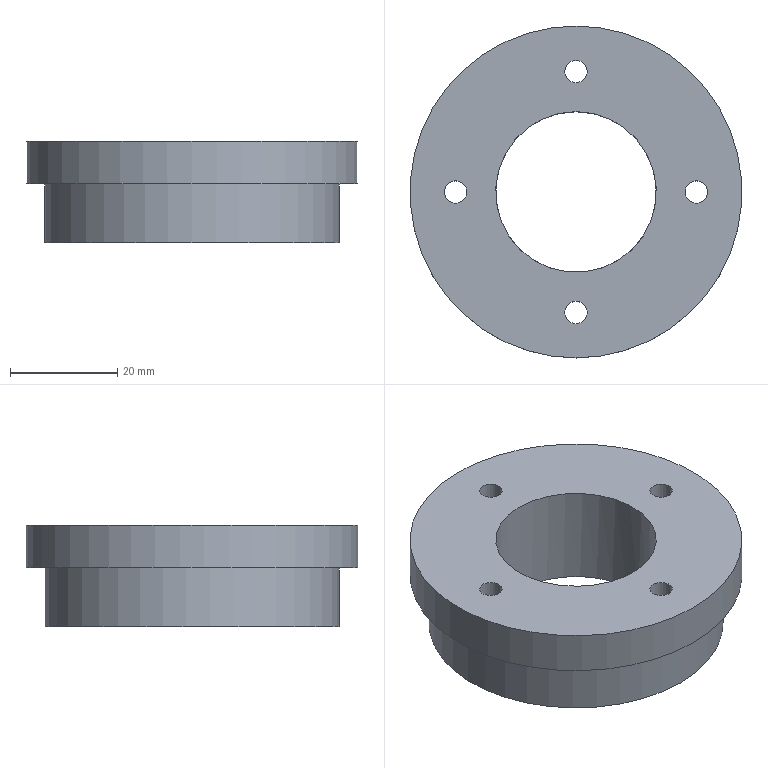Component | NX | FLANGE | 1 solid | 10 faces | box 62 x 62 x 19 mm | volume 35803 mm3 | cylinder 7 | plane 3 | commonest cylinder face diameters 4.2 x4 55 x1 62 x1 30 x1
STEP:
#1=CARTESIAN_POINT('',(0.,0.,0.));
#2=DIRECTION('',(0.,0.,1.));
#3=DIRECTION('',(1.,0.,0.));
#4=AXIS2_PLACEMENT_3D('',#1,#2,#3);
#5=CARTESIAN_POINT('',(0.,-27.5,14.));
#6=VERTEX_POINT('',#5);
#7=CARTESIAN_POINT('',(0.,0.,14.));
#8=DIRECTION('',(0.,0.,1.));
#9=DIRECTION('',(0.,-1.,0.));
#10=AXIS2_PLACEMENT_3D('',#7,#8,#9);
#11=CIRCLE('',#10,27.5);
#12=CARTESIAN_POINT('',(0.,0.,14.));
#13=DIRECTION('',(0.,0.,-1.));
#14=DIRECTION('',(0.,1.,0.));
#15=AXIS2_PLACEMENT_3D('',#12,#13,#14);
#16=CYLINDRICAL_SURFACE('',#15,27.5);
#17=CARTESIAN_POINT('',(9.425,0.));
#18=DIRECTION('',(-1.,0.));
#19=VECTOR('',#18,1.);
#20=LINE('',#17,#19);
#21=(GEOMETRIC_REPRESENTATION_CONTEXT(2)PARAMETRIC_REPRESENTATION_CONTEXT()REPRESENTATION_CONTEXT('',''));
#22=DEFINITIONAL_REPRESENTATION('',(#20),#21);
#23=PCURVE('',#16,#22);
#24=CARTESIAN_POINT('',(0.,0.,14.));
#25=DIRECTION('',(0.,0.,1.));
#26=DIRECTION('',(0.,-1.,0.));
#27=AXIS2_PLACEMENT_3D('',#24,#25,#26);
#28=PLANE('',#27);
#29=CARTESIAN_POINT('',(0.,0.));
#30=DIRECTION('',(1.,0.));
#31=AXIS2_PLACEMENT_2D('',#29,#30);
#32=CIRCLE('',#31,27.5);
#33=(GEOMETRIC_REPRESENTATION_CONTEXT(2)PARAMETRIC_REPRESENTATION_CONTEXT()REPRESENTATION_CONTEXT('',''));
#34=DEFINITIONAL_REPRESENTATION('',(#32),#33);
#35=PCURVE('',#28,#34);
#36=SURFACE_CURVE('',#11,(#23,#35),.PCURVE_S1.);
#37=EDGE_CURVE('',#6,#6,#36,.T.);
#38=ORIENTED_EDGE('',*,*,#37,.F.);
#39=CARTESIAN_POINT('',(0.,-27.5,3.));
#40=VERTEX_POINT('',#39);
#41=CARTESIAN_POINT('',(0.,-27.5,14.));
#42=CARTESIAN_POINT('',(0.,-27.5,3.));
#43=B_SPLINE_CURVE_WITH_KNOTS('',1,(#41,#42),.UNSPECIFIED.,.F.,.F.,(2,2),(0.,11.),.PIECEWISE_BEZIER_KNOTS.);
#44=CARTESIAN_POINT('',(9.425,0.));
#45=DIRECTION('',(0.,1.));
#46=VECTOR('',#45,1.);
#47=LINE('',#44,#46);
#48=(GEOMETRIC_REPRESENTATION_CONTEXT(2)PARAMETRIC_REPRESENTATION_CONTEXT()REPRESENTATION_CONTEXT('',''));
#49=DEFINITIONAL_REPRESENTATION('',(#47),#48);
#50=PCURVE('',#16,#49);
#51=CARTESIAN_POINT('',(3.142,0.));
#52=DIRECTION('',(0.,1.));
#53=VECTOR('',#52,1.);
#54=LINE('',#51,#53);
#55=(GEOMETRIC_REPRESENTATION_CONTEXT(2)PARAMETRIC_REPRESENTATION_CONTEXT()REPRESENTATION_CONTEXT('',''));
#56=DEFINITIONAL_REPRESENTATION('',(#54),#55);
#57=PCURVE('',#16,#56);
#58=SEAM_CURVE('',#43,(#50,#57),.PCURVE_S1.);
#59=EDGE_CURVE('',#6,#40,#58,.T.);
#60=ORIENTED_EDGE('',*,*,#59,.T.);
#61=CARTESIAN_POINT('',(0.,0.,3.));
#62=DIRECTION('',(0.,0.,1.));
#63=DIRECTION('',(0.,-1.,0.));
#64=AXIS2_PLACEMENT_3D('',#61,#62,#63);
#65=CIRCLE('',#64,27.5);
#66=CARTESIAN_POINT('',(9.425,11.));
#67=DIRECTION('',(-1.,0.));
#68=VECTOR('',#67,1.);
#69=LINE('',#66,#68);
#70=(GEOMETRIC_REPRESENTATION_CONTEXT(2)PARAMETRIC_REPRESENTATION_CONTEXT()REPRESENTATION_CONTEXT('',''));
#71=DEFINITIONAL_REPRESENTATION('',(#69),#70);
#72=PCURVE('',#16,#71);
#73=CARTESIAN_POINT('',(0.,0.,3.));
#74=DIRECTION('',(0.,0.,1.));
#75=DIRECTION('',(0.,-1.,0.));
#76=AXIS2_PLACEMENT_3D('',#73,#74,#75);
#77=PLANE('',#76);
#78=CARTESIAN_POINT('',(0.,0.));
#79=DIRECTION('',(1.,0.));
#80=AXIS2_PLACEMENT_2D('',#78,#79);
#81=CIRCLE('',#80,27.5);
#82=(GEOMETRIC_REPRESENTATION_CONTEXT(2)PARAMETRIC_REPRESENTATION_CONTEXT()REPRESENTATION_CONTEXT('',''));
#83=DEFINITIONAL_REPRESENTATION('',(#81),#82);
#84=PCURVE('',#77,#83);
#85=SURFACE_CURVE('',#65,(#72,#84),.PCURVE_S1.);
#86=EDGE_CURVE('',#40,#40,#85,.T.);
#87=ORIENTED_EDGE('',*,*,#86,.T.);
#88=ORIENTED_EDGE('',*,*,#59,.F.);
#89=EDGE_LOOP('',(#38,#60,#87,#88));
#90=FACE_BOUND('',#89,.T.);
#91=ADVANCED_FACE('',(#90),#16,.T.);
#92=CARTESIAN_POINT('',(0.,-24.6,3.));
#93=VERTEX_POINT('',#92);
#94=CARTESIAN_POINT('',(0.,-20.4,3.));
#95=VERTEX_POINT('',#94);
#96=CARTESIAN_POINT('',(0.,-22.5,3.));
#97=DIRECTION('',(0.,0.,1.));
#98=DIRECTION('',(0.,-1.,0.));
#99=AXIS2_PLACEMENT_3D('',#96,#97,#98);
#100=CIRCLE('',#99,2.1);
#101=CARTESIAN_POINT('',(22.5,0.));
#102=DIRECTION('',(1.,0.));
#103=AXIS2_PLACEMENT_2D('',#101,#102);
#104=CIRCLE('',#103,2.1);
#105=(GEOMETRIC_REPRESENTATION_CONTEXT(2)PARAMETRIC_REPRESENTATION_CONTEXT()REPRESENTATION_CONTEXT('',''));
#106=DEFINITIONAL_REPRESENTATION('',(#104),#105);
#107=PCURVE('',#77,#106);
#108=CARTESIAN_POINT('',(0.,-22.5,22.));
#109=DIRECTION('',(0.,0.,-1.));
#110=DIRECTION('',(0.,1.,0.));
#111=AXIS2_PLACEMENT_3D('',#108,#109,#110);
#112=CYLINDRICAL_SURFACE('',#111,2.1);
#113=CARTESIAN_POINT('',(3.142,19.));
#114=DIRECTION('',(-1.,0.));
#115=VECTOR('',#114,1.);
#116=LINE('',#113,#115);
#117=(GEOMETRIC_REPRESENTATION_CONTEXT(2)PARAMETRIC_REPRESENTATION_CONTEXT()REPRESENTATION_CONTEXT('',''));
#118=DEFINITIONAL_REPRESENTATION('',(#116),#117);
#119=PCURVE('',#112,#118);
#120=SURFACE_CURVE('',#100,(#107,#119),.PCURVE_S1.);
#121=EDGE_CURVE('',#93,#95,#120,.T.);
#122=ORIENTED_EDGE('',*,*,#121,.T.);
#123=CARTESIAN_POINT('',(0.,-22.5,3.));
#124=DIRECTION('',(0.,0.,1.));
#125=DIRECTION('',(0.,-1.,0.));
#126=AXIS2_PLACEMENT_3D('',#123,#124,#125);
#127=CIRCLE('',#126,2.1);
#128=CARTESIAN_POINT('',(22.5,0.));
#129=DIRECTION('',(1.,0.));
#130=AXIS2_PLACEMENT_2D('',#128,#129);
#131=CIRCLE('',#130,2.1);
#132=(GEOMETRIC_REPRESENTATION_CONTEXT(2)PARAMETRIC_REPRESENTATION_CONTEXT()REPRESENTATION_CONTEXT('',''));
#133=DEFINITIONAL_REPRESENTATION('',(#131),#132);
#134=PCURVE('',#77,#133);
#135=CARTESIAN_POINT('',(9.425,19.));
#136=DIRECTION('',(-1.,0.));
#137=VECTOR('',#136,1.);
#138=LINE('',#135,#137);
#139=(GEOMETRIC_REPRESENTATION_CONTEXT(2)PARAMETRIC_REPRESENTATION_CONTEXT()REPRESENTATION_CONTEXT('',''));
#140=DEFINITIONAL_REPRESENTATION('',(#138),#139);
#141=PCURVE('',#112,#140);
#142=SURFACE_CURVE('',#127,(#134,#141),.PCURVE_S1.);
#143=EDGE_CURVE('',#95,#93,#142,.T.);
#144=ORIENTED_EDGE('',*,*,#143,.T.);
#145=EDGE_LOOP('',(#122,#144));
#146=FACE_BOUND('',#145,.T.);
#147=CARTESIAN_POINT('',(22.5,-2.1,3.));
#148=VERTEX_POINT('',#147);
#149=CARTESIAN_POINT('',(22.5,2.1,3.));
#150=VERTEX_POINT('',#149);
#151=CARTESIAN_POINT('',(22.5,0.,3.));
#152=DIRECTION('',(0.,0.,1.));
#153=DIRECTION('',(0.,-1.,0.));
#154=AXIS2_PLACEMENT_3D('',#151,#152,#153);
#155=CIRCLE('',#154,2.1);
#156=CARTESIAN_POINT('',(0.,22.5));
#157=DIRECTION('',(1.,0.));
#158=AXIS2_PLACEMENT_2D('',#156,#157);
#159=CIRCLE('',#158,2.1);
#160=(GEOMETRIC_REPRESENTATION_CONTEXT(2)PARAMETRIC_REPRESENTATION_CONTEXT()REPRESENTATION_CONTEXT('',''));
#161=DEFINITIONAL_REPRESENTATION('',(#159),#160);
#162=PCURVE('',#77,#161);
#163=CARTESIAN_POINT('',(22.5,0.,22.));
#164=DIRECTION('',(0.,0.,-1.));
#165=DIRECTION('',(0.,1.,0.));
#166=AXIS2_PLACEMENT_3D('',#163,#164,#165);
#167=CYLINDRICAL_SURFACE('',#166,2.1);
#168=CARTESIAN_POINT('',(3.142,19.));
#169=DIRECTION('',(-1.,0.));
#170=VECTOR('',#169,1.);
#171=LINE('',#168,#170);
#172=(GEOMETRIC_REPRESENTATION_CONTEXT(2)PARAMETRIC_REPRESENTATION_CONTEXT()REPRESENTATION_CONTEXT('',''));
#173=DEFINITIONAL_REPRESENTATION('',(#171),#172);
#174=PCURVE('',#167,#173);
#175=SURFACE_CURVE('',#155,(#162,#174),.PCURVE_S1.);
#176=EDGE_CURVE('',#148,#150,#175,.T.);
#177=ORIENTED_EDGE('',*,*,#176,.T.);
#178=CARTESIAN_POINT('',(22.5,0.,3.));
#179=DIRECTION('',(0.,0.,1.));
#180=DIRECTION('',(0.,-1.,0.));
#181=AXIS2_PLACEMENT_3D('',#178,#179,#180);
#182=CIRCLE('',#181,2.1);
#183=CARTESIAN_POINT('',(0.,22.5));
#184=DIRECTION('',(1.,0.));
#185=AXIS2_PLACEMENT_2D('',#183,#184);
#186=CIRCLE('',#185,2.1);
#187=(GEOMETRIC_REPRESENTATION_CONTEXT(2)PARAMETRIC_REPRESENTATION_CONTEXT()REPRESENTATION_CONTEXT('',''));
#188=DEFINITIONAL_REPRESENTATION('',(#186),#187);
#189=PCURVE('',#77,#188);
#190=CARTESIAN_POINT('',(9.425,19.));
#191=DIRECTION('',(-1.,0.));
#192=VECTOR('',#191,1.);
#193=LINE('',#190,#192);
#194=(GEOMETRIC_REPRESENTATION_CONTEXT(2)PARAMETRIC_REPRESENTATION_CONTEXT()REPRESENTATION_CONTEXT('',''));
#195=DEFINITIONAL_REPRESENTATION('',(#193),#194);
#196=PCURVE('',#167,#195);
#197=SURFACE_CURVE('',#182,(#189,#196),.PCURVE_S1.);
#198=EDGE_CURVE('',#150,#148,#197,.T.);
#199=ORIENTED_EDGE('',*,*,#198,.T.);
#200=EDGE_LOOP('',(#177,#199));
#201=FACE_BOUND('',#200,.T.);
#202=CARTESIAN_POINT('',(-22.5,-2.1,3.));
#203=VERTEX_POINT('',#202);
#204=CARTESIAN_POINT('',(-22.5,2.1,3.));
#205=VERTEX_POINT('',#204);
#206=CARTESIAN_POINT('',(-22.5,0.,3.));
#207=DIRECTION('',(0.,0.,1.));
#208=DIRECTION('',(0.,-1.,0.));
#209=AXIS2_PLACEMENT_3D('',#206,#207,#208);
#210=CIRCLE('',#209,2.1);
#211=CARTESIAN_POINT('',(0.,-22.5));
#212=DIRECTION('',(1.,0.));
#213=AXIS2_PLACEMENT_2D('',#211,#212);
#214=CIRCLE('',#213,2.1);
#215=(GEOMETRIC_REPRESENTATION_CONTEXT(2)PARAMETRIC_REPRESENTATION_CONTEXT()REPRESENTATION_CONTEXT('',''));
#216=DEFINITIONAL_REPRESENTATION('',(#214),#215);
#217=PCURVE('',#77,#216);
#218=CARTESIAN_POINT('',(-22.5,0.,22.));
#219=DIRECTION('',(0.,0.,-1.));
#220=DIRECTION('',(0.,1.,0.));
#221=AXIS2_PLACEMENT_3D('',#218,#219,#220);
#222=CYLINDRICAL_SURFACE('',#221,2.1);
#223=CARTESIAN_POINT('',(3.142,19.));
#224=DIRECTION('',(-1.,0.));
#225=VECTOR('',#224,1.);
#226=LINE('',#223,#225);
#227=(GEOMETRIC_REPRESENTATION_CONTEXT(2)PARAMETRIC_REPRESENTATION_CONTEXT()REPRESENTATION_CONTEXT('',''));
#228=DEFINITIONAL_REPRESENTATION('',(#226),#227);
#229=PCURVE('',#222,#228);
#230=SURFACE_CURVE('',#210,(#217,#229),.PCURVE_S1.);
#231=EDGE_CURVE('',#203,#205,#230,.T.);
#232=ORIENTED_EDGE('',*,*,#231,.T.);
#233=CARTESIAN_POINT('',(-22.5,0.,3.));
#234=DIRECTION('',(0.,0.,1.));
#235=DIRECTION('',(0.,-1.,0.));
#236=AXIS2_PLACEMENT_3D('',#233,#234,#235);
#237=CIRCLE('',#236,2.1);
#238=CARTESIAN_POINT('',(0.,-22.5));
#239=DIRECTION('',(1.,0.));
#240=AXIS2_PLACEMENT_2D('',#238,#239);
#241=CIRCLE('',#240,2.1);
#242=(GEOMETRIC_REPRESENTATION_CONTEXT(2)PARAMETRIC_REPRESENTATION_CONTEXT()REPRESENTATION_CONTEXT('',''));
#243=DEFINITIONAL_REPRESENTATION('',(#241),#242);
#244=PCURVE('',#77,#243);
#245=CARTESIAN_POINT('',(9.425,19.));
#246=DIRECTION('',(-1.,0.));
#247=VECTOR('',#246,1.);
#248=LINE('',#245,#247);
#249=(GEOMETRIC_REPRESENTATION_CONTEXT(2)PARAMETRIC_REPRESENTATION_CONTEXT()REPRESENTATION_CONTEXT('',''));
#250=DEFINITIONAL_REPRESENTATION('',(#248),#249);
#251=PCURVE('',#222,#250);
#252=SURFACE_CURVE('',#237,(#244,#251),.PCURVE_S1.);
#253=EDGE_CURVE('',#205,#203,#252,.T.);
#254=ORIENTED_EDGE('',*,*,#253,.T.);
#255=EDGE_LOOP('',(#232,#254));
#256=FACE_BOUND('',#255,.T.);
#257=CARTESIAN_POINT('',(0.,20.4,3.));
#258=VERTEX_POINT('',#257);
#259=CARTESIAN_POINT('',(0.,24.6,3.));
#260=VERTEX_POINT('',#259);
#261=CARTESIAN_POINT('',(0.,22.5,3.));
#262=DIRECTION('',(0.,0.,1.));
#263=DIRECTION('',(0.,-1.,0.));
#264=AXIS2_PLACEMENT_3D('',#261,#262,#263);
#265=CIRCLE('',#264,2.1);
#266=CARTESIAN_POINT('',(-22.5,0.));
#267=DIRECTION('',(1.,0.));
#268=AXIS2_PLACEMENT_2D('',#266,#267);
#269=CIRCLE('',#268,2.1);
#270=(GEOMETRIC_REPRESENTATION_CONTEXT(2)PARAMETRIC_REPRESENTATION_CONTEXT()REPRESENTATION_CONTEXT('',''));
#271=DEFINITIONAL_REPRESENTATION('',(#269),#270);
#272=PCURVE('',#77,#271);
#273=CARTESIAN_POINT('',(0.,22.5,22.));
#274=DIRECTION('',(0.,0.,-1.));
#275=DIRECTION('',(0.,1.,0.));
#276=AXIS2_PLACEMENT_3D('',#273,#274,#275);
#277=CYLINDRICAL_SURFACE('',#276,2.1);
#278=CARTESIAN_POINT('',(3.142,19.));
#279=DIRECTION('',(-1.,0.));
#280=VECTOR('',#279,1.);
#281=LINE('',#278,#280);
#282=(GEOMETRIC_REPRESENTATION_CONTEXT(2)PARAMETRIC_REPRESENTATION_CONTEXT()REPRESENTATION_CONTEXT('',''));
#283=DEFINITIONAL_REPRESENTATION('',(#281),#282);
#284=PCURVE('',#277,#283);
#285=SURFACE_CURVE('',#265,(#272,#284),.PCURVE_S1.);
#286=EDGE_CURVE('',#258,#260,#285,.T.);
#287=ORIENTED_EDGE('',*,*,#286,.T.);
#288=CARTESIAN_POINT('',(0.,22.5,3.));
#289=DIRECTION('',(0.,0.,1.));
#290=DIRECTION('',(0.,-1.,0.));
#291=AXIS2_PLACEMENT_3D('',#288,#289,#290);
#292=CIRCLE('',#291,2.1);
#293=CARTESIAN_POINT('',(-22.5,0.));
#294=DIRECTION('',(1.,0.));
#295=AXIS2_PLACEMENT_2D('',#293,#294);
#296=CIRCLE('',#295,2.1);
#297=(GEOMETRIC_REPRESENTATION_CONTEXT(2)PARAMETRIC_REPRESENTATION_CONTEXT()REPRESENTATION_CONTEXT('',''));
#298=DEFINITIONAL_REPRESENTATION('',(#296),#297);
#299=PCURVE('',#77,#298);
#300=CARTESIAN_POINT('',(9.425,19.));
#301=DIRECTION('',(-1.,0.));
#302=VECTOR('',#301,1.);
#303=LINE('',#300,#302);
#304=(GEOMETRIC_REPRESENTATION_CONTEXT(2)PARAMETRIC_REPRESENTATION_CONTEXT()REPRESENTATION_CONTEXT('',''));
#305=DEFINITIONAL_REPRESENTATION('',(#303),#304);
#306=PCURVE('',#277,#305);
#307=SURFACE_CURVE('',#292,(#299,#306),.PCURVE_S1.);
#308=EDGE_CURVE('',#260,#258,#307,.T.);
#309=ORIENTED_EDGE('',*,*,#308,.T.);
#310=EDGE_LOOP('',(#287,#309));
#311=FACE_BOUND('',#310,.T.);
#312=CARTESIAN_POINT('',(0.,-15.,3.));
#313=VERTEX_POINT('',#312);
#314=CARTESIAN_POINT('',(0.,15.,3.));
#315=VERTEX_POINT('',#314);
#316=CARTESIAN_POINT('',(0.,0.,3.));
#317=DIRECTION('',(0.,0.,1.));
#318=DIRECTION('',(0.,-1.,0.));
#319=AXIS2_PLACEMENT_3D('',#316,#317,#318);
#320=CIRCLE('',#319,15.);
#321=CARTESIAN_POINT('',(0.,0.));
#322=DIRECTION('',(1.,0.));
#323=AXIS2_PLACEMENT_2D('',#321,#322);
#324=CIRCLE('',#323,15.);
#325=(GEOMETRIC_REPRESENTATION_CONTEXT(2)PARAMETRIC_REPRESENTATION_CONTEXT()REPRESENTATION_CONTEXT('',''));
#326=DEFINITIONAL_REPRESENTATION('',(#324),#325);
#327=PCURVE('',#77,#326);
#328=CARTESIAN_POINT('',(0.,0.,22.));
#329=DIRECTION('',(0.,0.,-1.));
#330=DIRECTION('',(0.,1.,0.));
#331=AXIS2_PLACEMENT_3D('',#328,#329,#330);
#332=CYLINDRICAL_SURFACE('',#331,15.);
#333=CARTESIAN_POINT('',(3.142,19.));
#334=DIRECTION('',(-1.,0.));
#335=VECTOR('',#334,1.);
#336=LINE('',#333,#335);
#337=(GEOMETRIC_REPRESENTATION_CONTEXT(2)PARAMETRIC_REPRESENTATION_CONTEXT()REPRESENTATION_CONTEXT('',''));
#338=DEFINITIONAL_REPRESENTATION('',(#336),#337);
#339=PCURVE('',#332,#338);
#340=SURFACE_CURVE('',#320,(#327,#339),.PCURVE_S1.);
#341=EDGE_CURVE('',#313,#315,#340,.T.);
#342=ORIENTED_EDGE('',*,*,#341,.T.);
#343=CARTESIAN_POINT('',(0.,0.,3.));
#344=DIRECTION('',(0.,0.,1.));
#345=DIRECTION('',(0.,-1.,0.));
#346=AXIS2_PLACEMENT_3D('',#343,#344,#345);
#347=CIRCLE('',#346,15.);
#348=CARTESIAN_POINT('',(0.,0.));
#349=DIRECTION('',(1.,0.));
#350=AXIS2_PLACEMENT_2D('',#348,#349);
#351=CIRCLE('',#350,15.);
#352=(GEOMETRIC_REPRESENTATION_CONTEXT(2)PARAMETRIC_REPRESENTATION_CONTEXT()REPRESENTATION_CONTEXT('',''));
#353=DEFINITIONAL_REPRESENTATION('',(#351),#352);
#354=PCURVE('',#77,#353);
#355=CARTESIAN_POINT('',(9.425,19.));
#356=DIRECTION('',(-1.,0.));
#357=VECTOR('',#356,1.);
#358=LINE('',#355,#357);
#359=(GEOMETRIC_REPRESENTATION_CONTEXT(2)PARAMETRIC_REPRESENTATION_CONTEXT()REPRESENTATION_CONTEXT('',''));
#360=DEFINITIONAL_REPRESENTATION('',(#358),#359);
#361=PCURVE('',#332,#360);
#362=SURFACE_CURVE('',#347,(#354,#361),.PCURVE_S1.);
#363=EDGE_CURVE('',#315,#313,#362,.T.);
#364=ORIENTED_EDGE('',*,*,#363,.T.);
#365=EDGE_LOOP('',(#342,#364));
#366=FACE_BOUND('',#365,.T.);
#367=ORIENTED_EDGE('',*,*,#86,.F.);
#368=EDGE_LOOP('',(#367));
#369=FACE_BOUND('',#368,.T.);
#370=ADVANCED_FACE('',(#146,#201,#256,#311,#366,#369),#77,.F.);
#371=CARTESIAN_POINT('',(0.,-31.,22.));
#372=VERTEX_POINT('',#371);
#373=CARTESIAN_POINT('',(0.,0.,22.));
#374=DIRECTION('',(0.,0.,1.));
#375=DIRECTION('',(0.,-1.,0.));
#376=AXIS2_PLACEMENT_3D('',#373,#374,#375);
#377=CIRCLE('',#376,31.);
#378=CARTESIAN_POINT('',(0.,0.,22.));
#379=DIRECTION('',(0.,0.,-1.));
#380=DIRECTION('',(0.,1.,0.));
#381=AXIS2_PLACEMENT_3D('',#378,#379,#380);
#382=CYLINDRICAL_SURFACE('',#381,31.);
#383=CARTESIAN_POINT('',(9.425,0.));
#384=DIRECTION('',(-1.,0.));
#385=VECTOR('',#384,1.);
#386=LINE('',#383,#385);
#387=(GEOMETRIC_REPRESENTATION_CONTEXT(2)PARAMETRIC_REPRESENTATION_CONTEXT()REPRESENTATION_CONTEXT('',''));
#388=DEFINITIONAL_REPRESENTATION('',(#386),#387);
#389=PCURVE('',#382,#388);
#390=CARTESIAN_POINT('',(0.,0.,22.));
#391=DIRECTION('',(0.,0.,1.));
#392=DIRECTION('',(0.,-1.,0.));
#393=AXIS2_PLACEMENT_3D('',#390,#391,#392);
#394=PLANE('',#393);
#395=CARTESIAN_POINT('',(0.,0.));
#396=DIRECTION('',(1.,0.));
#397=AXIS2_PLACEMENT_2D('',#395,#396);
#398=CIRCLE('',#397,31.);
#399=(GEOMETRIC_REPRESENTATION_CONTEXT(2)PARAMETRIC_REPRESENTATION_CONTEXT()REPRESENTATION_CONTEXT('',''));
#400=DEFINITIONAL_REPRESENTATION('',(#398),#399);
#401=PCURVE('',#394,#400);
#402=SURFACE_CURVE('',#377,(#389,#401),.PCURVE_S1.);
#403=EDGE_CURVE('',#372,#372,#402,.T.);
#404=ORIENTED_EDGE('',*,*,#403,.F.);
#405=CARTESIAN_POINT('',(0.,-31.,14.));
#406=VERTEX_POINT('',#405);
#407=CARTESIAN_POINT('',(0.,-31.,22.));
#408=CARTESIAN_POINT('',(0.,-31.,14.));
#409=B_SPLINE_CURVE_WITH_KNOTS('',1,(#407,#408),.UNSPECIFIED.,.F.,.F.,(2,2),(0.,8.),.PIECEWISE_BEZIER_KNOTS.);
#410=CARTESIAN_POINT('',(9.425,0.));
#411=DIRECTION('',(0.,1.));
#412=VECTOR('',#411,1.);
#413=LINE('',#410,#412);
#414=(GEOMETRIC_REPRESENTATION_CONTEXT(2)PARAMETRIC_REPRESENTATION_CONTEXT()REPRESENTATION_CONTEXT('',''));
#415=DEFINITIONAL_REPRESENTATION('',(#413),#414);
#416=PCURVE('',#382,#415);
#417=CARTESIAN_POINT('',(3.142,0.));
#418=DIRECTION('',(0.,1.));
#419=VECTOR('',#418,1.);
#420=LINE('',#417,#419);
#421=(GEOMETRIC_REPRESENTATION_CONTEXT(2)PARAMETRIC_REPRESENTATION_CONTEXT()REPRESENTATION_CONTEXT('',''));
#422=DEFINITIONAL_REPRESENTATION('',(#420),#421);
#423=PCURVE('',#382,#422);
#424=SEAM_CURVE('',#409,(#416,#423),.PCURVE_S1.);
#425=EDGE_CURVE('',#372,#406,#424,.T.);
#426=ORIENTED_EDGE('',*,*,#425,.T.);
#427=CARTESIAN_POINT('',(0.,0.,14.));
#428=DIRECTION('',(0.,0.,1.));
#429=DIRECTION('',(0.,-1.,0.));
#430=AXIS2_PLACEMENT_3D('',#427,#428,#429);
#431=CIRCLE('',#430,31.);
#432=CARTESIAN_POINT('',(9.425,8.));
#433=DIRECTION('',(-1.,0.));
#434=VECTOR('',#433,1.);
#435=LINE('',#432,#434);
#436=(GEOMETRIC_REPRESENTATION_CONTEXT(2)PARAMETRIC_REPRESENTATION_CONTEXT()REPRESENTATION_CONTEXT('',''));
#437=DEFINITIONAL_REPRESENTATION('',(#435),#436);
#438=PCURVE('',#382,#437);
#439=CARTESIAN_POINT('',(0.,0.));
#440=DIRECTION('',(1.,0.));
#441=AXIS2_PLACEMENT_2D('',#439,#440);
#442=CIRCLE('',#441,31.);
#443=(GEOMETRIC_REPRESENTATION_CONTEXT(2)PARAMETRIC_REPRESENTATION_CONTEXT()REPRESENTATION_CONTEXT('',''));
#444=DEFINITIONAL_REPRESENTATION('',(#442),#443);
#445=PCURVE('',#28,#444);
#446=SURFACE_CURVE('',#431,(#438,#445),.PCURVE_S1.);
#447=EDGE_CURVE('',#406,#406,#446,.T.);
#448=ORIENTED_EDGE('',*,*,#447,.T.);
#449=ORIENTED_EDGE('',*,*,#425,.F.);
#450=EDGE_LOOP('',(#404,#426,#448,#449));
#451=FACE_BOUND('',#450,.T.);
#452=ADVANCED_FACE('',(#451),#382,.T.);
#453=CARTESIAN_POINT('',(0.,-20.4,22.));
#454=VERTEX_POINT('',#453);
#455=CARTESIAN_POINT('',(0.,-22.5,22.));
#456=DIRECTION('',(0.,0.,-1.));
#457=DIRECTION('',(0.,1.,0.));
#458=AXIS2_PLACEMENT_3D('',#455,#456,#457);
#459=CIRCLE('',#458,2.1);
#460=CARTESIAN_POINT('',(20.4,0.));
#461=CARTESIAN_POINT('',(20.4,3.637));
#462=CARTESIAN_POINT('',(23.55,1.819));
#463=CARTESIAN_POINT('',(26.7,0.));
#464=CARTESIAN_POINT('',(23.55,-1.819));
#465=CARTESIAN_POINT('',(20.4,-3.637));
#466=CARTESIAN_POINT('',(20.4,0.));
#467=(BOUNDED_CURVE()B_SPLINE_CURVE(2,(#460,#461,#462,#463,#464,#465,#466),.UNSPECIFIED.,.T.,.F.)B_SPLINE_CURVE_WITH_KNOTS((1,2,2,2,2,1),(-2.094,0.,2.094,4.189,6.283,8.378),.UNSPECIFIED.)CURVE()GEOMETRIC_REPRESENTATION_ITEM()RATIONAL_B_SPLINE_CURVE((1.,0.5,1.,0.5,1.,0.5,1.))REPRESENTATION_ITEM(''));
#468=(GEOMETRIC_REPRESENTATION_CONTEXT(2)PARAMETRIC_REPRESENTATION_CONTEXT()REPRESENTATION_CONTEXT('',''));
#469=DEFINITIONAL_REPRESENTATION('',(#467),#468);
#470=PCURVE('',#394,#469);
#471=CARTESIAN_POINT('',(0.,0.));
#472=DIRECTION('',(1.,0.));
#473=VECTOR('',#472,1.);
#474=LINE('',#471,#473);
#475=(GEOMETRIC_REPRESENTATION_CONTEXT(2)PARAMETRIC_REPRESENTATION_CONTEXT()REPRESENTATION_CONTEXT('',''));
#476=DEFINITIONAL_REPRESENTATION('',(#474),#475);
#477=PCURVE('',#112,#476);
#478=SURFACE_CURVE('',#459,(#470,#477),.PCURVE_S1.);
#479=EDGE_CURVE('',#454,#454,#478,.T.);
#480=ORIENTED_EDGE('',*,*,#479,.T.);
#481=EDGE_LOOP('',(#480));
#482=FACE_BOUND('',#481,.T.);
#483=CARTESIAN_POINT('',(22.5,2.1,22.));
#484=VERTEX_POINT('',#483);
#485=CARTESIAN_POINT('',(22.5,0.,22.));
#486=DIRECTION('',(0.,0.,-1.));
#487=DIRECTION('',(0.,1.,0.));
#488=AXIS2_PLACEMENT_3D('',#485,#486,#487);
#489=CIRCLE('',#488,2.1);
#490=CARTESIAN_POINT('',(-2.1,22.5));
#491=CARTESIAN_POINT('',(-2.1,26.137));
#492=CARTESIAN_POINT('',(1.05,24.319));
#493=CARTESIAN_POINT('',(4.2,22.5));
#494=CARTESIAN_POINT('',(1.05,20.681));
#495=CARTESIAN_POINT('',(-2.1,18.863));
#496=CARTESIAN_POINT('',(-2.1,22.5));
#497=(BOUNDED_CURVE()B_SPLINE_CURVE(2,(#490,#491,#492,#493,#494,#495,#496),.UNSPECIFIED.,.T.,.F.)B_SPLINE_CURVE_WITH_KNOTS((1,2,2,2,2,1),(-2.094,0.,2.094,4.189,6.283,8.378),.UNSPECIFIED.)CURVE()GEOMETRIC_REPRESENTATION_ITEM()RATIONAL_B_SPLINE_CURVE((1.,0.5,1.,0.5,1.,0.5,1.))REPRESENTATION_ITEM(''));
#498=(GEOMETRIC_REPRESENTATION_CONTEXT(2)PARAMETRIC_REPRESENTATION_CONTEXT()REPRESENTATION_CONTEXT('',''));
#499=DEFINITIONAL_REPRESENTATION('',(#497),#498);
#500=PCURVE('',#394,#499);
#501=CARTESIAN_POINT('',(0.,0.));
#502=DIRECTION('',(1.,0.));
#503=VECTOR('',#502,1.);
#504=LINE('',#501,#503);
#505=(GEOMETRIC_REPRESENTATION_CONTEXT(2)PARAMETRIC_REPRESENTATION_CONTEXT()REPRESENTATION_CONTEXT('',''));
#506=DEFINITIONAL_REPRESENTATION('',(#504),#505);
#507=PCURVE('',#167,#506);
#508=SURFACE_CURVE('',#489,(#500,#507),.PCURVE_S1.);
#509=EDGE_CURVE('',#484,#484,#508,.T.);
#510=ORIENTED_EDGE('',*,*,#509,.T.);
#511=EDGE_LOOP('',(#510));
#512=FACE_BOUND('',#511,.T.);
#513=CARTESIAN_POINT('',(-22.5,2.1,22.));
#514=VERTEX_POINT('',#513);
#515=CARTESIAN_POINT('',(-22.5,0.,22.));
#516=DIRECTION('',(0.,0.,-1.));
#517=DIRECTION('',(0.,1.,0.));
#518=AXIS2_PLACEMENT_3D('',#515,#516,#517);
#519=CIRCLE('',#518,2.1);
#520=CARTESIAN_POINT('',(-2.1,-22.5));
#521=CARTESIAN_POINT('',(-2.1,-18.863));
#522=CARTESIAN_POINT('',(1.05,-20.681));
#523=CARTESIAN_POINT('',(4.2,-22.5));
#524=CARTESIAN_POINT('',(1.05,-24.319));
#525=CARTESIAN_POINT('',(-2.1,-26.137));
#526=CARTESIAN_POINT('',(-2.1,-22.5));
#527=(BOUNDED_CURVE()B_SPLINE_CURVE(2,(#520,#521,#522,#523,#524,#525,#526),.UNSPECIFIED.,.T.,.F.)B_SPLINE_CURVE_WITH_KNOTS((1,2,2,2,2,1),(-2.094,0.,2.094,4.189,6.283,8.378),.UNSPECIFIED.)CURVE()GEOMETRIC_REPRESENTATION_ITEM()RATIONAL_B_SPLINE_CURVE((1.,0.5,1.,0.5,1.,0.5,1.))REPRESENTATION_ITEM(''));
#528=(GEOMETRIC_REPRESENTATION_CONTEXT(2)PARAMETRIC_REPRESENTATION_CONTEXT()REPRESENTATION_CONTEXT('',''));
#529=DEFINITIONAL_REPRESENTATION('',(#527),#528);
#530=PCURVE('',#394,#529);
#531=CARTESIAN_POINT('',(0.,0.));
#532=DIRECTION('',(1.,0.));
#533=VECTOR('',#532,1.);
#534=LINE('',#531,#533);
#535=(GEOMETRIC_REPRESENTATION_CONTEXT(2)PARAMETRIC_REPRESENTATION_CONTEXT()REPRESENTATION_CONTEXT('',''));
#536=DEFINITIONAL_REPRESENTATION('',(#534),#535);
#537=PCURVE('',#222,#536);
#538=SURFACE_CURVE('',#519,(#530,#537),.PCURVE_S1.);
#539=EDGE_CURVE('',#514,#514,#538,.T.);
#540=ORIENTED_EDGE('',*,*,#539,.T.);
#541=EDGE_LOOP('',(#540));
#542=FACE_BOUND('',#541,.T.);
#543=CARTESIAN_POINT('',(0.,24.6,22.));
#544=VERTEX_POINT('',#543);
#545=CARTESIAN_POINT('',(0.,22.5,22.));
#546=DIRECTION('',(0.,0.,-1.));
#547=DIRECTION('',(0.,1.,0.));
#548=AXIS2_PLACEMENT_3D('',#545,#546,#547);
#549=CIRCLE('',#548,2.1);
#550=CARTESIAN_POINT('',(-24.6,0.));
#551=CARTESIAN_POINT('',(-24.6,3.637));
#552=CARTESIAN_POINT('',(-21.45,1.819));
#553=CARTESIAN_POINT('',(-18.3,0.));
#554=CARTESIAN_POINT('',(-21.45,-1.819));
#555=CARTESIAN_POINT('',(-24.6,-3.637));
#556=CARTESIAN_POINT('',(-24.6,0.));
#557=(BOUNDED_CURVE()B_SPLINE_CURVE(2,(#550,#551,#552,#553,#554,#555,#556),.UNSPECIFIED.,.T.,.F.)B_SPLINE_CURVE_WITH_KNOTS((1,2,2,2,2,1),(-2.094,0.,2.094,4.189,6.283,8.378),.UNSPECIFIED.)CURVE()GEOMETRIC_REPRESENTATION_ITEM()RATIONAL_B_SPLINE_CURVE((1.,0.5,1.,0.5,1.,0.5,1.))REPRESENTATION_ITEM(''));
#558=(GEOMETRIC_REPRESENTATION_CONTEXT(2)PARAMETRIC_REPRESENTATION_CONTEXT()REPRESENTATION_CONTEXT('',''));
#559=DEFINITIONAL_REPRESENTATION('',(#557),#558);
#560=PCURVE('',#394,#559);
#561=CARTESIAN_POINT('',(0.,0.));
#562=DIRECTION('',(1.,0.));
#563=VECTOR('',#562,1.);
#564=LINE('',#561,#563);
#565=(GEOMETRIC_REPRESENTATION_CONTEXT(2)PARAMETRIC_REPRESENTATION_CONTEXT()REPRESENTATION_CONTEXT('',''));
#566=DEFINITIONAL_REPRESENTATION('',(#564),#565);
#567=PCURVE('',#277,#566);
#568=SURFACE_CURVE('',#549,(#560,#567),.PCURVE_S1.);
#569=EDGE_CURVE('',#544,#544,#568,.T.);
#570=ORIENTED_EDGE('',*,*,#569,.T.);
#571=EDGE_LOOP('',(#570));
#572=FACE_BOUND('',#571,.T.);
#573=CARTESIAN_POINT('',(0.,15.,22.));
#574=VERTEX_POINT('',#573);
#575=CARTESIAN_POINT('',(0.,0.,22.));
#576=DIRECTION('',(0.,0.,-1.));
#577=DIRECTION('',(0.,1.,0.));
#578=AXIS2_PLACEMENT_3D('',#575,#576,#577);
#579=CIRCLE('',#578,15.);
#580=CARTESIAN_POINT('',(-15.,0.));
#581=CARTESIAN_POINT('',(-15.,25.981));
#582=CARTESIAN_POINT('',(7.5,12.99));
#583=CARTESIAN_POINT('',(30.,0.));
#584=CARTESIAN_POINT('',(7.5,-12.99));
#585=CARTESIAN_POINT('',(-15.,-25.981));
#586=CARTESIAN_POINT('',(-15.,0.));
#587=(BOUNDED_CURVE()B_SPLINE_CURVE(2,(#580,#581,#582,#583,#584,#585,#586),.UNSPECIFIED.,.T.,.F.)B_SPLINE_CURVE_WITH_KNOTS((1,2,2,2,2,1),(-2.094,0.,2.094,4.189,6.283,8.378),.UNSPECIFIED.)CURVE()GEOMETRIC_REPRESENTATION_ITEM()RATIONAL_B_SPLINE_CURVE((1.,0.5,1.,0.5,1.,0.5,1.))REPRESENTATION_ITEM(''));
#588=(GEOMETRIC_REPRESENTATION_CONTEXT(2)PARAMETRIC_REPRESENTATION_CONTEXT()REPRESENTATION_CONTEXT('',''));
#589=DEFINITIONAL_REPRESENTATION('',(#587),#588);
#590=PCURVE('',#394,#589);
#591=CARTESIAN_POINT('',(0.,0.));
#592=DIRECTION('',(1.,0.));
#593=VECTOR('',#592,1.);
#594=LINE('',#591,#593);
#595=(GEOMETRIC_REPRESENTATION_CONTEXT(2)PARAMETRIC_REPRESENTATION_CONTEXT()REPRESENTATION_CONTEXT('',''));
#596=DEFINITIONAL_REPRESENTATION('',(#594),#595);
#597=PCURVE('',#332,#596);
#598=SURFACE_CURVE('',#579,(#590,#597),.PCURVE_S1.);
#599=EDGE_CURVE('',#574,#574,#598,.T.);
#600=ORIENTED_EDGE('',*,*,#599,.T.);
#601=EDGE_LOOP('',(#600));
#602=FACE_BOUND('',#601,.T.);
#603=ORIENTED_EDGE('',*,*,#403,.T.);
#604=EDGE_LOOP('',(#603));
#605=FACE_BOUND('',#604,.T.);
#606=ADVANCED_FACE('',(#482,#512,#542,#572,#602,#605),#394,.T.);
#607=ORIENTED_EDGE('',*,*,#37,.T.);
#608=EDGE_LOOP('',(#607));
#609=FACE_BOUND('',#608,.T.);
#610=ORIENTED_EDGE('',*,*,#447,.F.);
#611=EDGE_LOOP('',(#610));
#612=FACE_BOUND('',#611,.T.);
#613=ADVANCED_FACE('',(#609,#612),#28,.F.);
#614=ORIENTED_EDGE('',*,*,#599,.T.);
#615=CARTESIAN_POINT('',(0.,15.,22.));
#616=CARTESIAN_POINT('',(0.,15.,3.));
#617=B_SPLINE_CURVE_WITH_KNOTS('',1,(#615,#616),.UNSPECIFIED.,.F.,.F.,(2,2),(0.,19.),.PIECEWISE_BEZIER_KNOTS.);
#618=CARTESIAN_POINT('',(6.283,0.));
#619=DIRECTION('',(0.,1.));
#620=VECTOR('',#619,1.);
#621=LINE('',#618,#620);
#622=(GEOMETRIC_REPRESENTATION_CONTEXT(2)PARAMETRIC_REPRESENTATION_CONTEXT()REPRESENTATION_CONTEXT('',''));
#623=DEFINITIONAL_REPRESENTATION('',(#621),#622);
#624=PCURVE('',#332,#623);
#625=CARTESIAN_POINT('',(0.,0.));
#626=DIRECTION('',(0.,1.));
#627=VECTOR('',#626,1.);
#628=LINE('',#625,#627);
#629=(GEOMETRIC_REPRESENTATION_CONTEXT(2)PARAMETRIC_REPRESENTATION_CONTEXT()REPRESENTATION_CONTEXT('',''));
#630=DEFINITIONAL_REPRESENTATION('',(#628),#629);
#631=PCURVE('',#332,#630);
#632=SEAM_CURVE('',#617,(#624,#631),.PCURVE_S1.);
#633=EDGE_CURVE('',#574,#315,#632,.T.);
#634=ORIENTED_EDGE('',*,*,#633,.T.);
#635=ORIENTED_EDGE('',*,*,#363,.T.);
#636=ORIENTED_EDGE('',*,*,#341,.T.);
#637=ORIENTED_EDGE('',*,*,#633,.F.);
#638=EDGE_LOOP('',(#614,#634,#635,#636,#637));
#639=FACE_BOUND('',#638,.F.);
#640=ADVANCED_FACE('',(#639),#332,.F.);
#641=ORIENTED_EDGE('',*,*,#569,.T.);
#642=CARTESIAN_POINT('',(0.,24.6,22.));
#643=CARTESIAN_POINT('',(0.,24.6,3.));
#644=B_SPLINE_CURVE_WITH_KNOTS('',1,(#642,#643),.UNSPECIFIED.,.F.,.F.,(2,2),(0.,19.),.PIECEWISE_BEZIER_KNOTS.);
#645=CARTESIAN_POINT('',(6.283,0.));
#646=DIRECTION('',(0.,1.));
#647=VECTOR('',#646,1.);
#648=LINE('',#645,#647);
#649=(GEOMETRIC_REPRESENTATION_CONTEXT(2)PARAMETRIC_REPRESENTATION_CONTEXT()REPRESENTATION_CONTEXT('',''));
#650=DEFINITIONAL_REPRESENTATION('',(#648),#649);
#651=PCURVE('',#277,#650);
#652=CARTESIAN_POINT('',(0.,0.));
#653=DIRECTION('',(0.,1.));
#654=VECTOR('',#653,1.);
#655=LINE('',#652,#654);
#656=(GEOMETRIC_REPRESENTATION_CONTEXT(2)PARAMETRIC_REPRESENTATION_CONTEXT()REPRESENTATION_CONTEXT('',''));
#657=DEFINITIONAL_REPRESENTATION('',(#655),#656);
#658=PCURVE('',#277,#657);
#659=SEAM_CURVE('',#644,(#651,#658),.PCURVE_S1.);
#660=EDGE_CURVE('',#544,#260,#659,.T.);
#661=ORIENTED_EDGE('',*,*,#660,.T.);
#662=ORIENTED_EDGE('',*,*,#308,.T.);
#663=ORIENTED_EDGE('',*,*,#286,.T.);
#664=ORIENTED_EDGE('',*,*,#660,.F.);
#665=EDGE_LOOP('',(#641,#661,#662,#663,#664));
#666=FACE_BOUND('',#665,.F.);
#667=ADVANCED_FACE('',(#666),#277,.F.);
#668=ORIENTED_EDGE('',*,*,#539,.T.);
#669=CARTESIAN_POINT('',(-22.5,2.1,22.));
#670=CARTESIAN_POINT('',(-22.5,2.1,3.));
#671=B_SPLINE_CURVE_WITH_KNOTS('',1,(#669,#670),.UNSPECIFIED.,.F.,.F.,(2,2),(0.,19.),.PIECEWISE_BEZIER_KNOTS.);
#672=CARTESIAN_POINT('',(6.283,0.));
#673=DIRECTION('',(0.,1.));
#674=VECTOR('',#673,1.);
#675=LINE('',#672,#674);
#676=(GEOMETRIC_REPRESENTATION_CONTEXT(2)PARAMETRIC_REPRESENTATION_CONTEXT()REPRESENTATION_CONTEXT('',''));
#677=DEFINITIONAL_REPRESENTATION('',(#675),#676);
#678=PCURVE('',#222,#677);
#679=CARTESIAN_POINT('',(0.,0.));
#680=DIRECTION('',(0.,1.));
#681=VECTOR('',#680,1.);
#682=LINE('',#679,#681);
#683=(GEOMETRIC_REPRESENTATION_CONTEXT(2)PARAMETRIC_REPRESENTATION_CONTEXT()REPRESENTATION_CONTEXT('',''));
#684=DEFINITIONAL_REPRESENTATION('',(#682),#683);
#685=PCURVE('',#222,#684);
#686=SEAM_CURVE('',#671,(#678,#685),.PCURVE_S1.);
#687=EDGE_CURVE('',#514,#205,#686,.T.);
#688=ORIENTED_EDGE('',*,*,#687,.T.);
#689=ORIENTED_EDGE('',*,*,#253,.T.);
#690=ORIENTED_EDGE('',*,*,#231,.T.);
#691=ORIENTED_EDGE('',*,*,#687,.F.);
#692=EDGE_LOOP('',(#668,#688,#689,#690,#691));
#693=FACE_BOUND('',#692,.F.);
#694=ADVANCED_FACE('',(#693),#222,.F.);
#695=ORIENTED_EDGE('',*,*,#509,.T.);
#696=CARTESIAN_POINT('',(22.5,2.1,22.));
#697=CARTESIAN_POINT('',(22.5,2.1,3.));
#698=B_SPLINE_CURVE_WITH_KNOTS('',1,(#696,#697),.UNSPECIFIED.,.F.,.F.,(2,2),(0.,19.),.PIECEWISE_BEZIER_KNOTS.);
#699=CARTESIAN_POINT('',(6.283,0.));
#700=DIRECTION('',(0.,1.));
#701=VECTOR('',#700,1.);
#702=LINE('',#699,#701);
#703=(GEOMETRIC_REPRESENTATION_CONTEXT(2)PARAMETRIC_REPRESENTATION_CONTEXT()REPRESENTATION_CONTEXT('',''));
#704=DEFINITIONAL_REPRESENTATION('',(#702),#703);
#705=PCURVE('',#167,#704);
#706=CARTESIAN_POINT('',(0.,0.));
#707=DIRECTION('',(0.,1.));
#708=VECTOR('',#707,1.);
#709=LINE('',#706,#708);
#710=(GEOMETRIC_REPRESENTATION_CONTEXT(2)PARAMETRIC_REPRESENTATION_CONTEXT()REPRESENTATION_CONTEXT('',''));
#711=DEFINITIONAL_REPRESENTATION('',(#709),#710);
#712=PCURVE('',#167,#711);
#713=SEAM_CURVE('',#698,(#705,#712),.PCURVE_S1.);
#714=EDGE_CURVE('',#484,#150,#713,.T.);
#715=ORIENTED_EDGE('',*,*,#714,.T.);
#716=ORIENTED_EDGE('',*,*,#198,.T.);
#717=ORIENTED_EDGE('',*,*,#176,.T.);
#718=ORIENTED_EDGE('',*,*,#714,.F.);
#719=EDGE_LOOP('',(#695,#715,#716,#717,#718));
#720=FACE_BOUND('',#719,.F.);
#721=ADVANCED_FACE('',(#720),#167,.F.);
#722=ORIENTED_EDGE('',*,*,#479,.T.);
#723=CARTESIAN_POINT('',(0.,-20.4,22.));
#724=CARTESIAN_POINT('',(0.,-20.4,3.));
#725=B_SPLINE_CURVE_WITH_KNOTS('',1,(#723,#724),.UNSPECIFIED.,.F.,.F.,(2,2),(0.,19.),.PIECEWISE_BEZIER_KNOTS.);
#726=CARTESIAN_POINT('',(6.283,0.));
#727=DIRECTION('',(0.,1.));
#728=VECTOR('',#727,1.);
#729=LINE('',#726,#728);
#730=(GEOMETRIC_REPRESENTATION_CONTEXT(2)PARAMETRIC_REPRESENTATION_CONTEXT()REPRESENTATION_CONTEXT('',''));
#731=DEFINITIONAL_REPRESENTATION('',(#729),#730);
#732=PCURVE('',#112,#731);
#733=CARTESIAN_POINT('',(0.,0.));
#734=DIRECTION('',(0.,1.));
#735=VECTOR('',#734,1.);
#736=LINE('',#733,#735);
#737=(GEOMETRIC_REPRESENTATION_CONTEXT(2)PARAMETRIC_REPRESENTATION_CONTEXT()REPRESENTATION_CONTEXT('',''));
#738=DEFINITIONAL_REPRESENTATION('',(#736),#737);
#739=PCURVE('',#112,#738);
#740=SEAM_CURVE('',#725,(#732,#739),.PCURVE_S1.);
#741=EDGE_CURVE('',#454,#95,#740,.T.);
#742=ORIENTED_EDGE('',*,*,#741,.T.);
#743=ORIENTED_EDGE('',*,*,#143,.T.);
#744=ORIENTED_EDGE('',*,*,#121,.T.);
#745=ORIENTED_EDGE('',*,*,#741,.F.);
#746=EDGE_LOOP('',(#722,#742,#743,#744,#745));
#747=FACE_BOUND('',#746,.F.);
#748=ADVANCED_FACE('',(#747),#112,.F.);
#749=CLOSED_SHELL('',(#91,#370,#452,#606,#613,#640,#667,#694,#721,#748));
#750=MANIFOLD_SOLID_BREP('',#749);
#751=(LENGTH_UNIT()NAMED_UNIT(*)SI_UNIT(.MILLI.,.METRE.));
#752=UNCERTAINTY_MEASURE_WITH_UNIT(LENGTH_MEASURE(0.000005),#751,'','');
#753=(NAMED_UNIT(*)PLANE_ANGLE_UNIT()SI_UNIT($,.RADIAN.));
#754=(NAMED_UNIT(*)SI_UNIT($,.STERADIAN.)SOLID_ANGLE_UNIT());
#755=(GEOMETRIC_REPRESENTATION_CONTEXT(3)GLOBAL_UNCERTAINTY_ASSIGNED_CONTEXT((#752))GLOBAL_UNIT_ASSIGNED_CONTEXT((#751,#753,#754))REPRESENTATION_CONTEXT('',''));
#756=ADVANCED_BREP_SHAPE_REPRESENTATION('',(#4,#750),#755);